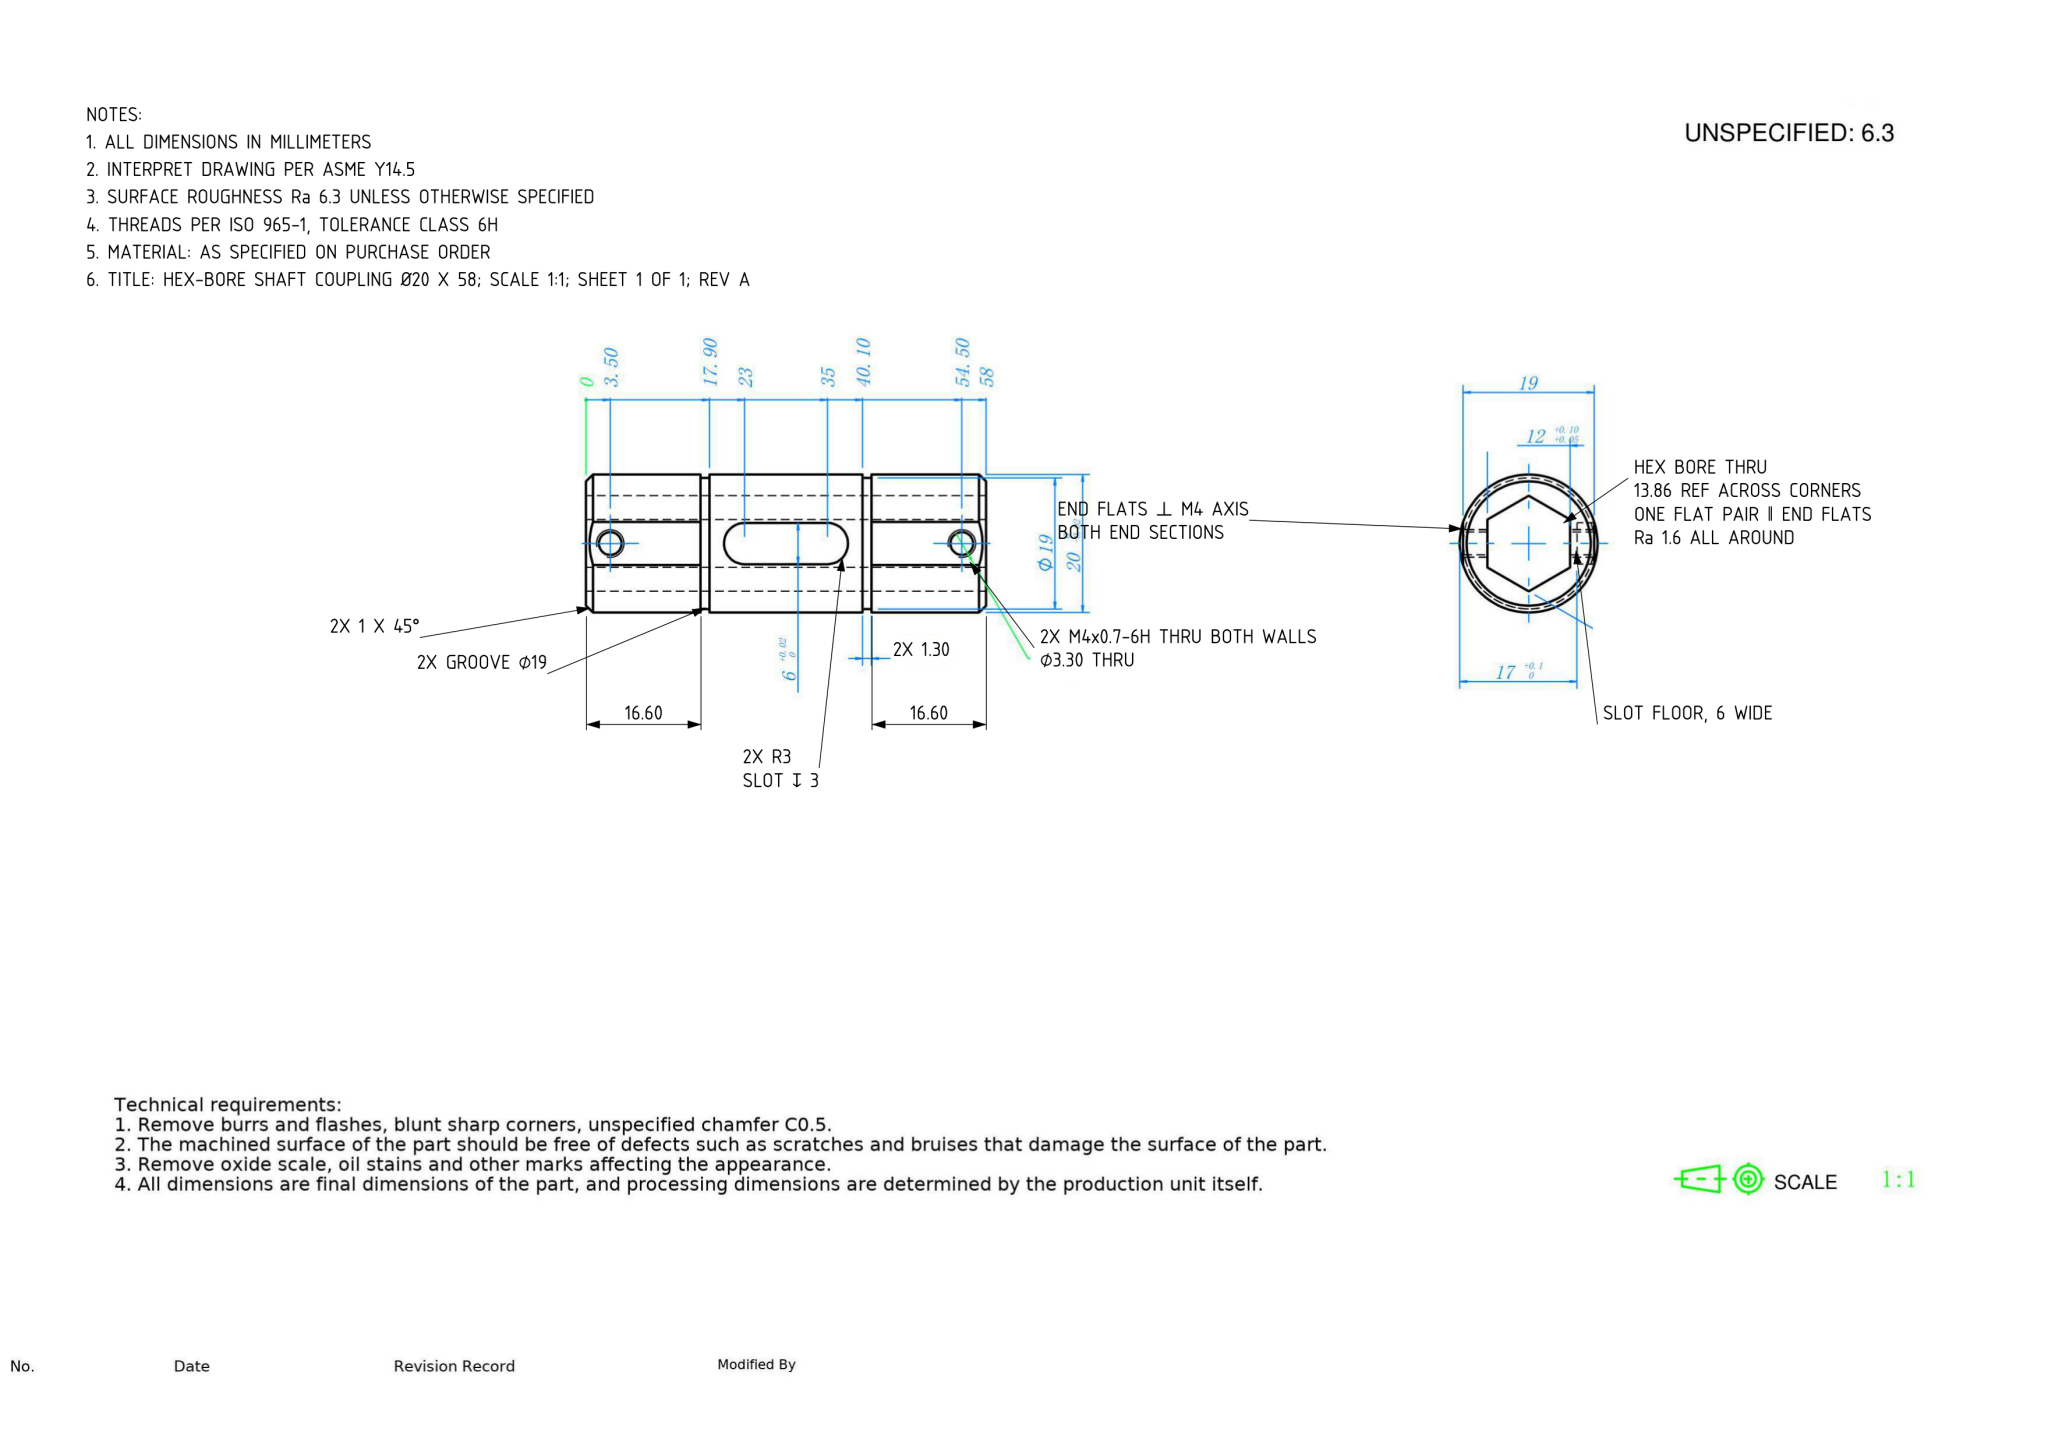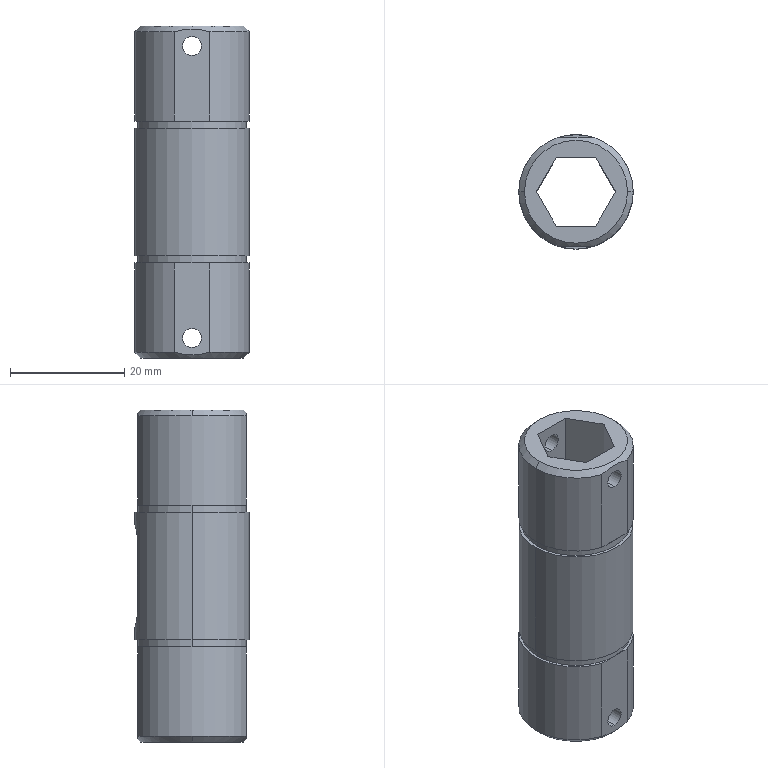Part | NX | mm | 1 solid | 48 faces | box 20 x 20 x 58 mm | volume 10309 mm3 | cylinder 23 | plane 21 | cone 4 | commonest cylinder face diameters 3.3 x8 20 x8 19 x4 6 x3